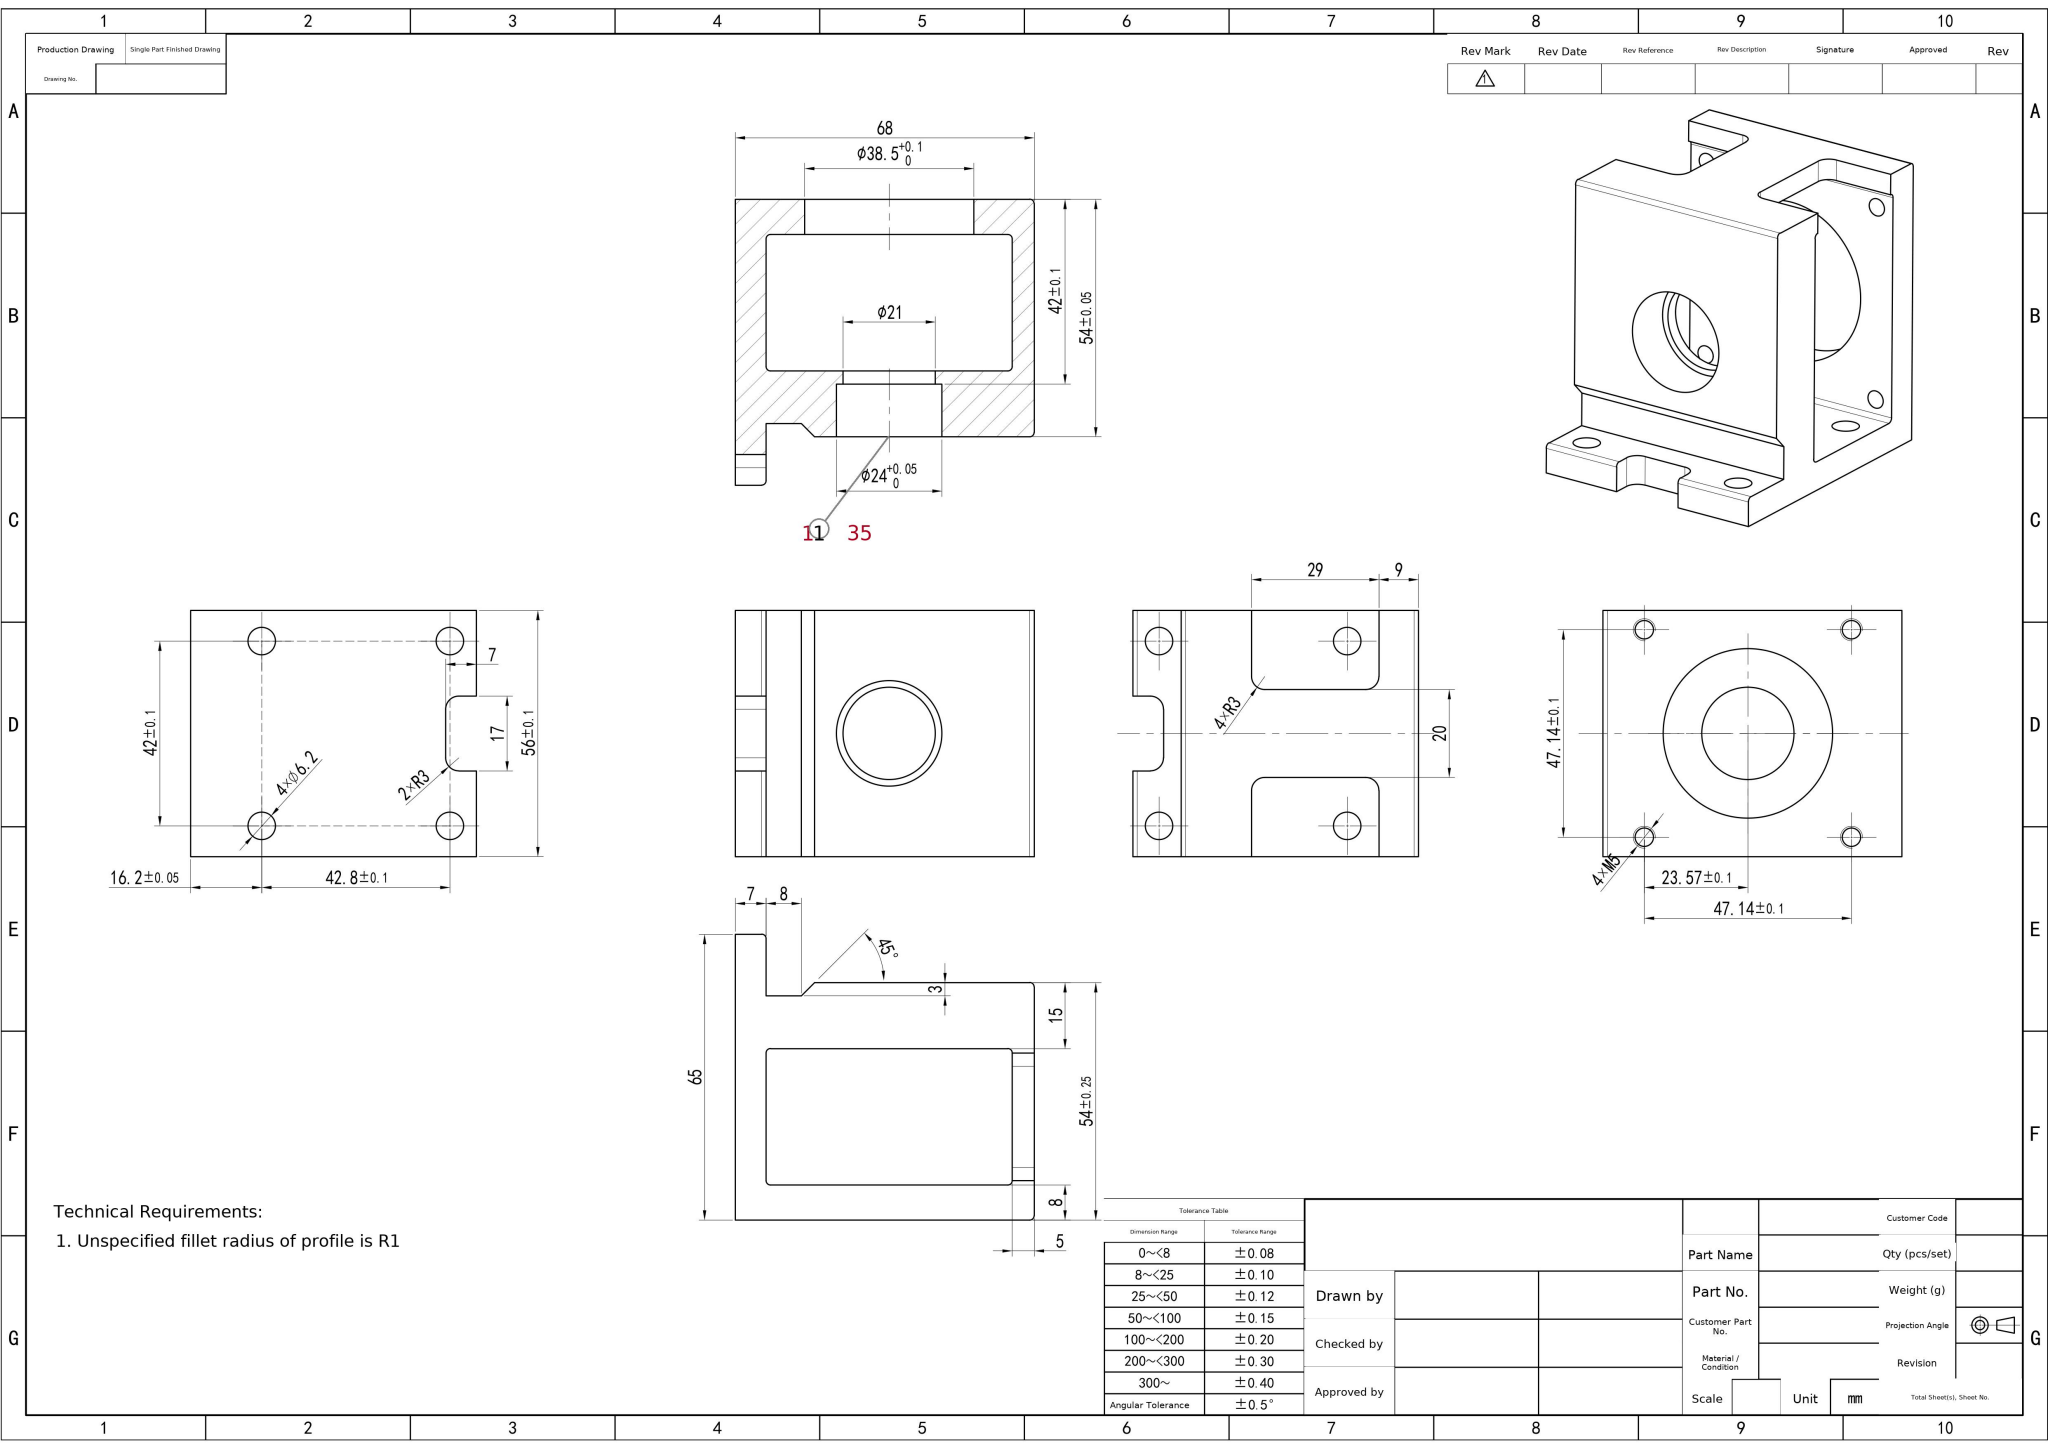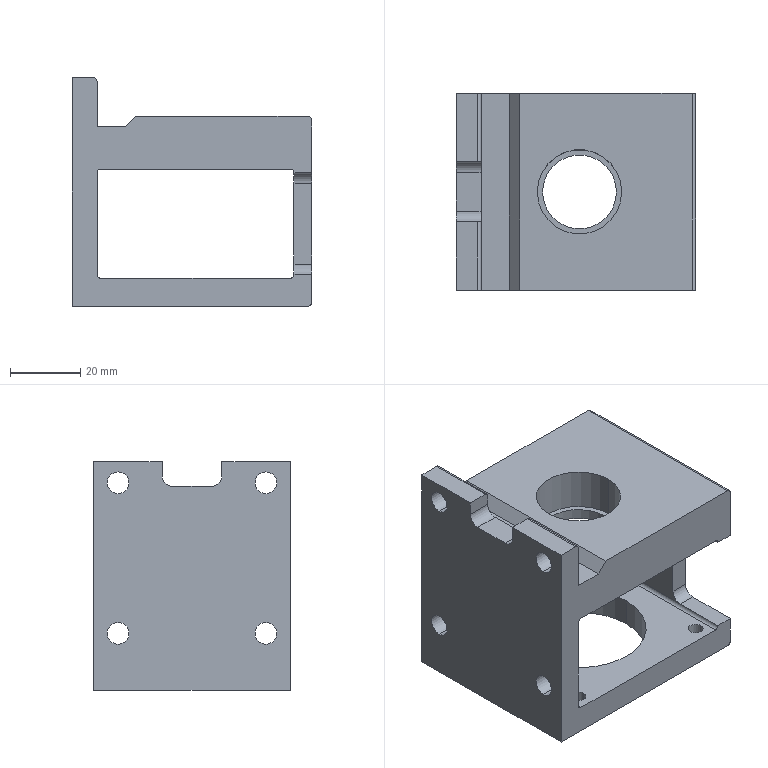Part | SolidWorks | mm | 1 solid | 61 faces | box 68 x 56 x 65 mm | volume 88091 mm3 | cylinder 36 | plane 25 | commonest cylinder face diameters 6.2 x8 4.2 x8 2 x8 6 x6 38.5 x2 24 x2 21 x2